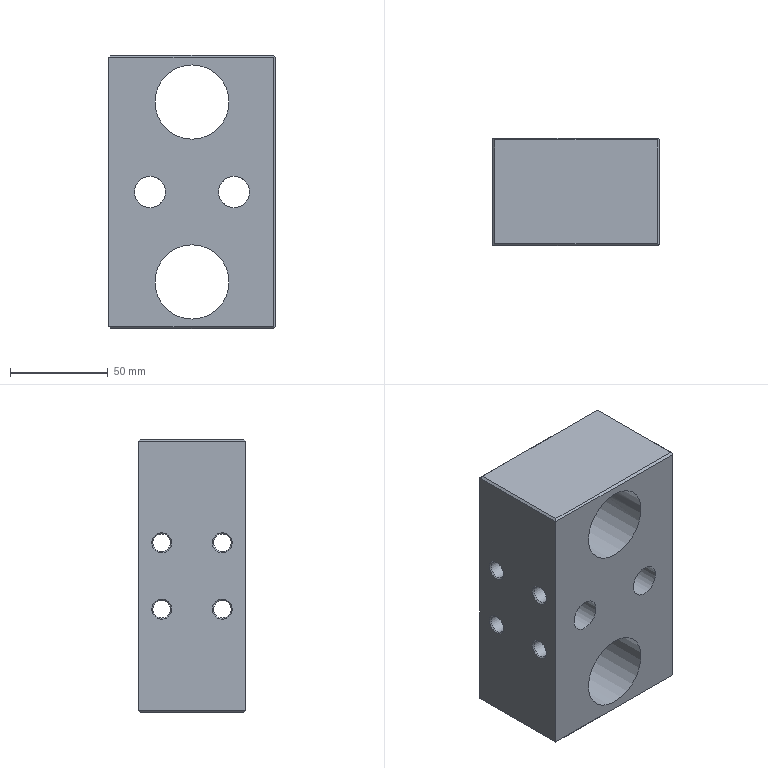Component | NX | YMSR_PET_P04 | 1 solid | 46 faces | volume 480651 mm3 | plane 20 | cylinder 13 | cone 13 | commonest cylinder face diameters 9 x4 15 x4 38 x2 16 x2 6.8 x1